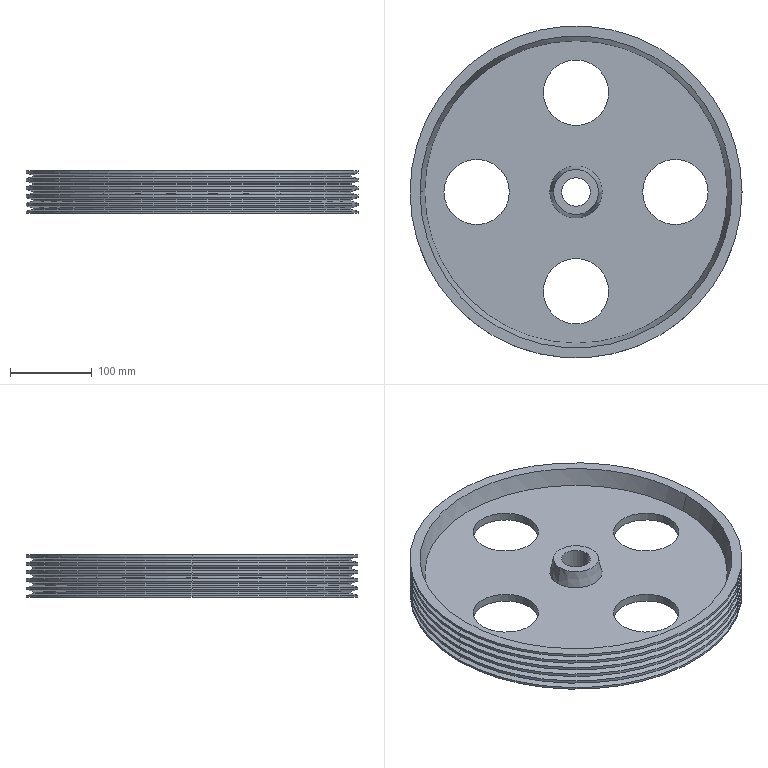Component | SolidWorks | Pulley-1 | 1 solid | 66 faces | box 406 x 406 x 52 mm | volume 1721003 mm3 | cylinder 32 | cone 28 | plane 6 | commonest cylinder face diameters 406 x12 390 x10 80 x8 35 x2
build123d program:
from build123d import *

# Parameters (mm, degrees)
SKETCH2_R          = 40
CUT_EXTRUDE3_DEPTH = 455.979


with BuildPart() as part:
    # Sketch1 → Revolve1 (revolve)
    with BuildSketch(Plane(origin=(0, 0, 0), x_dir=(0, 0, -1), z_dir=(1, 0, 0)), mode=Mode.PRIVATE) as revolve1_sk:
        Polygon((0, 0), (3, 0), (5.144, -8), (7.391, -8), (9.535, 0), (13, 0), (15.144, -8), (17.391, -8), (19.535, 0), (23, 0), (25.144, -8), (27.391, -8), (29.535, 0), (33, 0), (35.144, -8), (37.391, -8), (39.535, 0), (43, 0), (45.144, -8), (47.391, -8), (49.535, 0), (52, 0), (52, -12.289), (31, -18), (31, -171), (52, -175.467), (52, -185.5), (0, -185.5), (0, -175.467), (21, -171), (21, -18), (0, -12.289), align=None)
    revolve(revolve1_sk.sketch.rotate(Axis((0, -203, -52), (0, 0, 1)), 90), axis=Axis((0, -203, -52), (0, 0, 1)))

    # Sketch2 → Cut-Extrude3 (cut, through all)
    with BuildSketch(Plane(origin=(0, 0, -31), x_dir=(-1, 0, 0), z_dir=(0, 0, -1))):
        with Locations((0, -81.5)):
            Circle(SKETCH2_R)
        with Locations((121.5, -203)):
            Circle(SKETCH2_R)
        with Locations((0, -324.5)):
            Circle(SKETCH2_R)
        with Locations((-121.5, -203)):
            Circle(SKETCH2_R)
    extrude(amount=-CUT_EXTRUDE3_DEPTH, mode=Mode.SUBTRACT)


solid = part.part

# Placed as in the assembly
solid = solid.moved(Location((35.733, 218.31, 121.5), (0, 0, 0)))